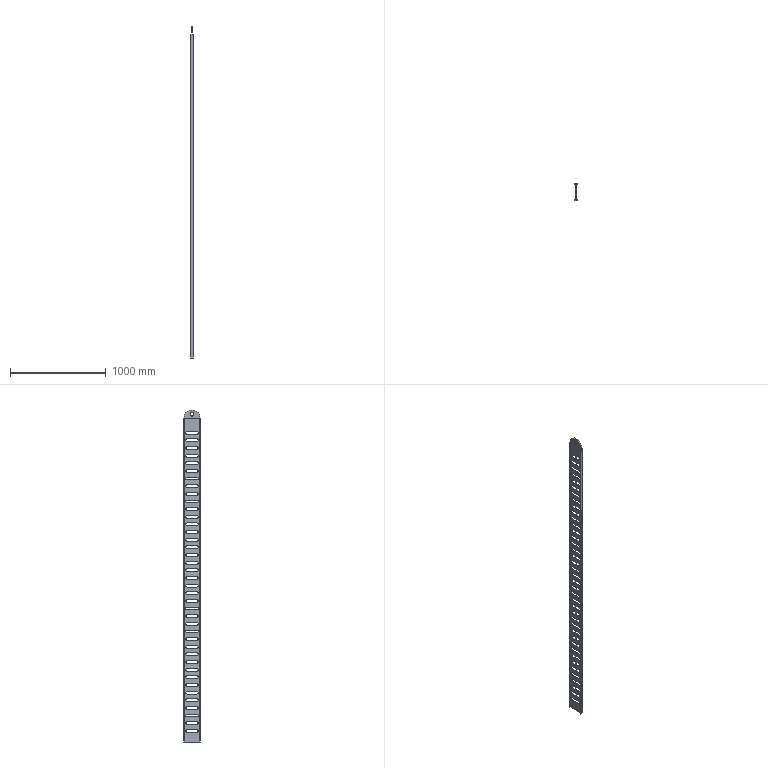Component | NX | FRONT_BEAM | 1 solid | 181 faces | volume 2387392 mm3 | plane 99 | cylinder 82 | commonest cylinder face diameters 30 x80 170 x1 40 x1